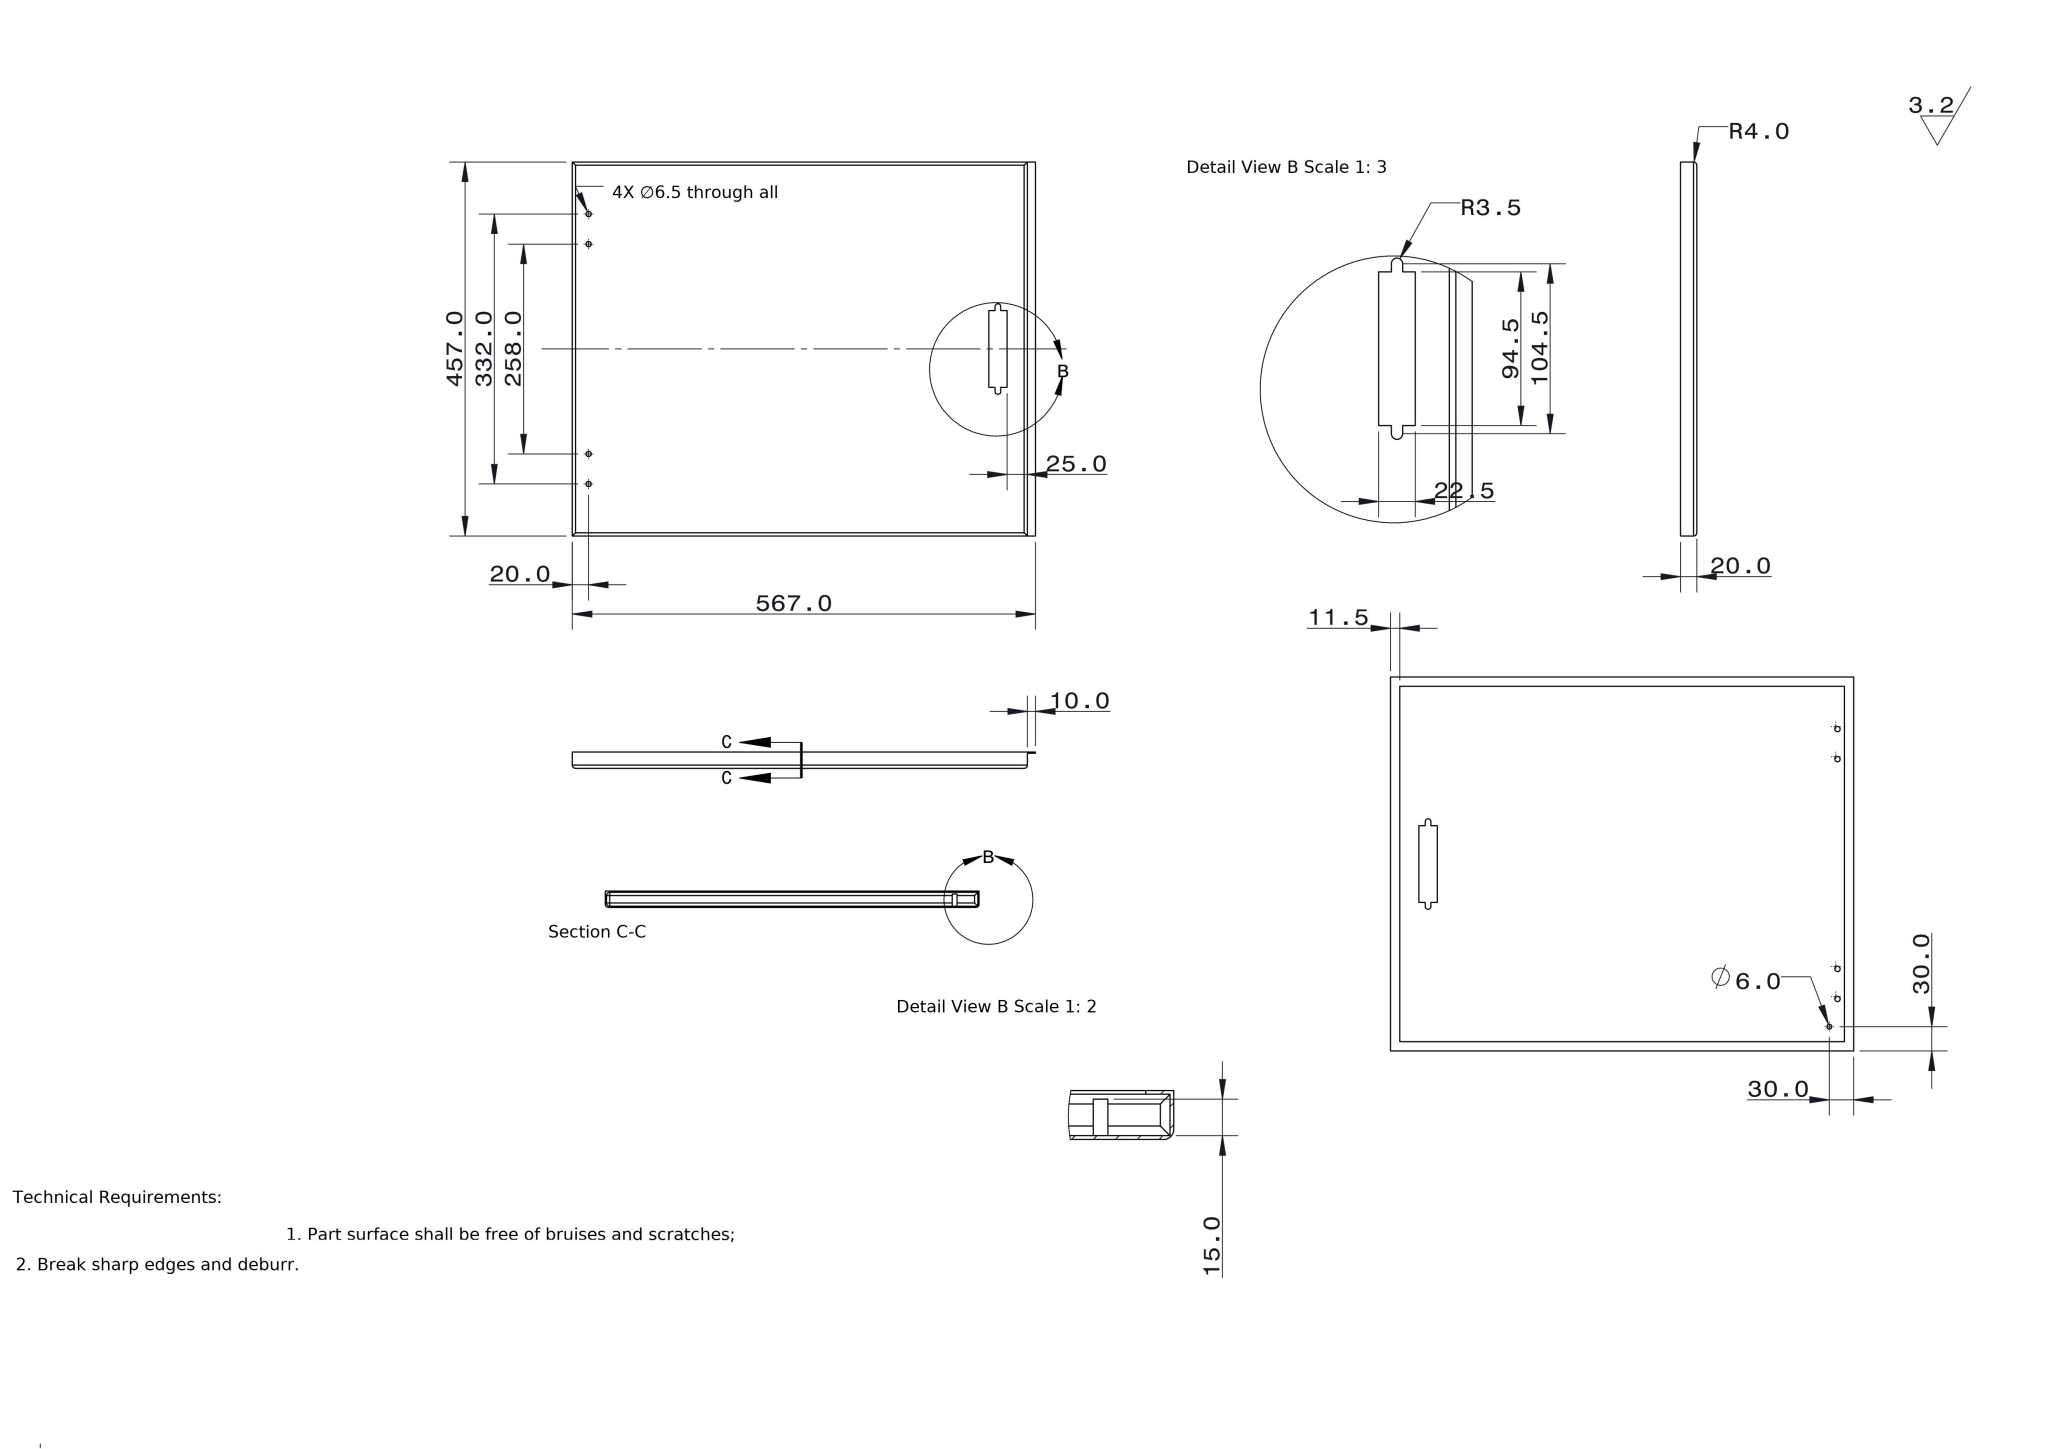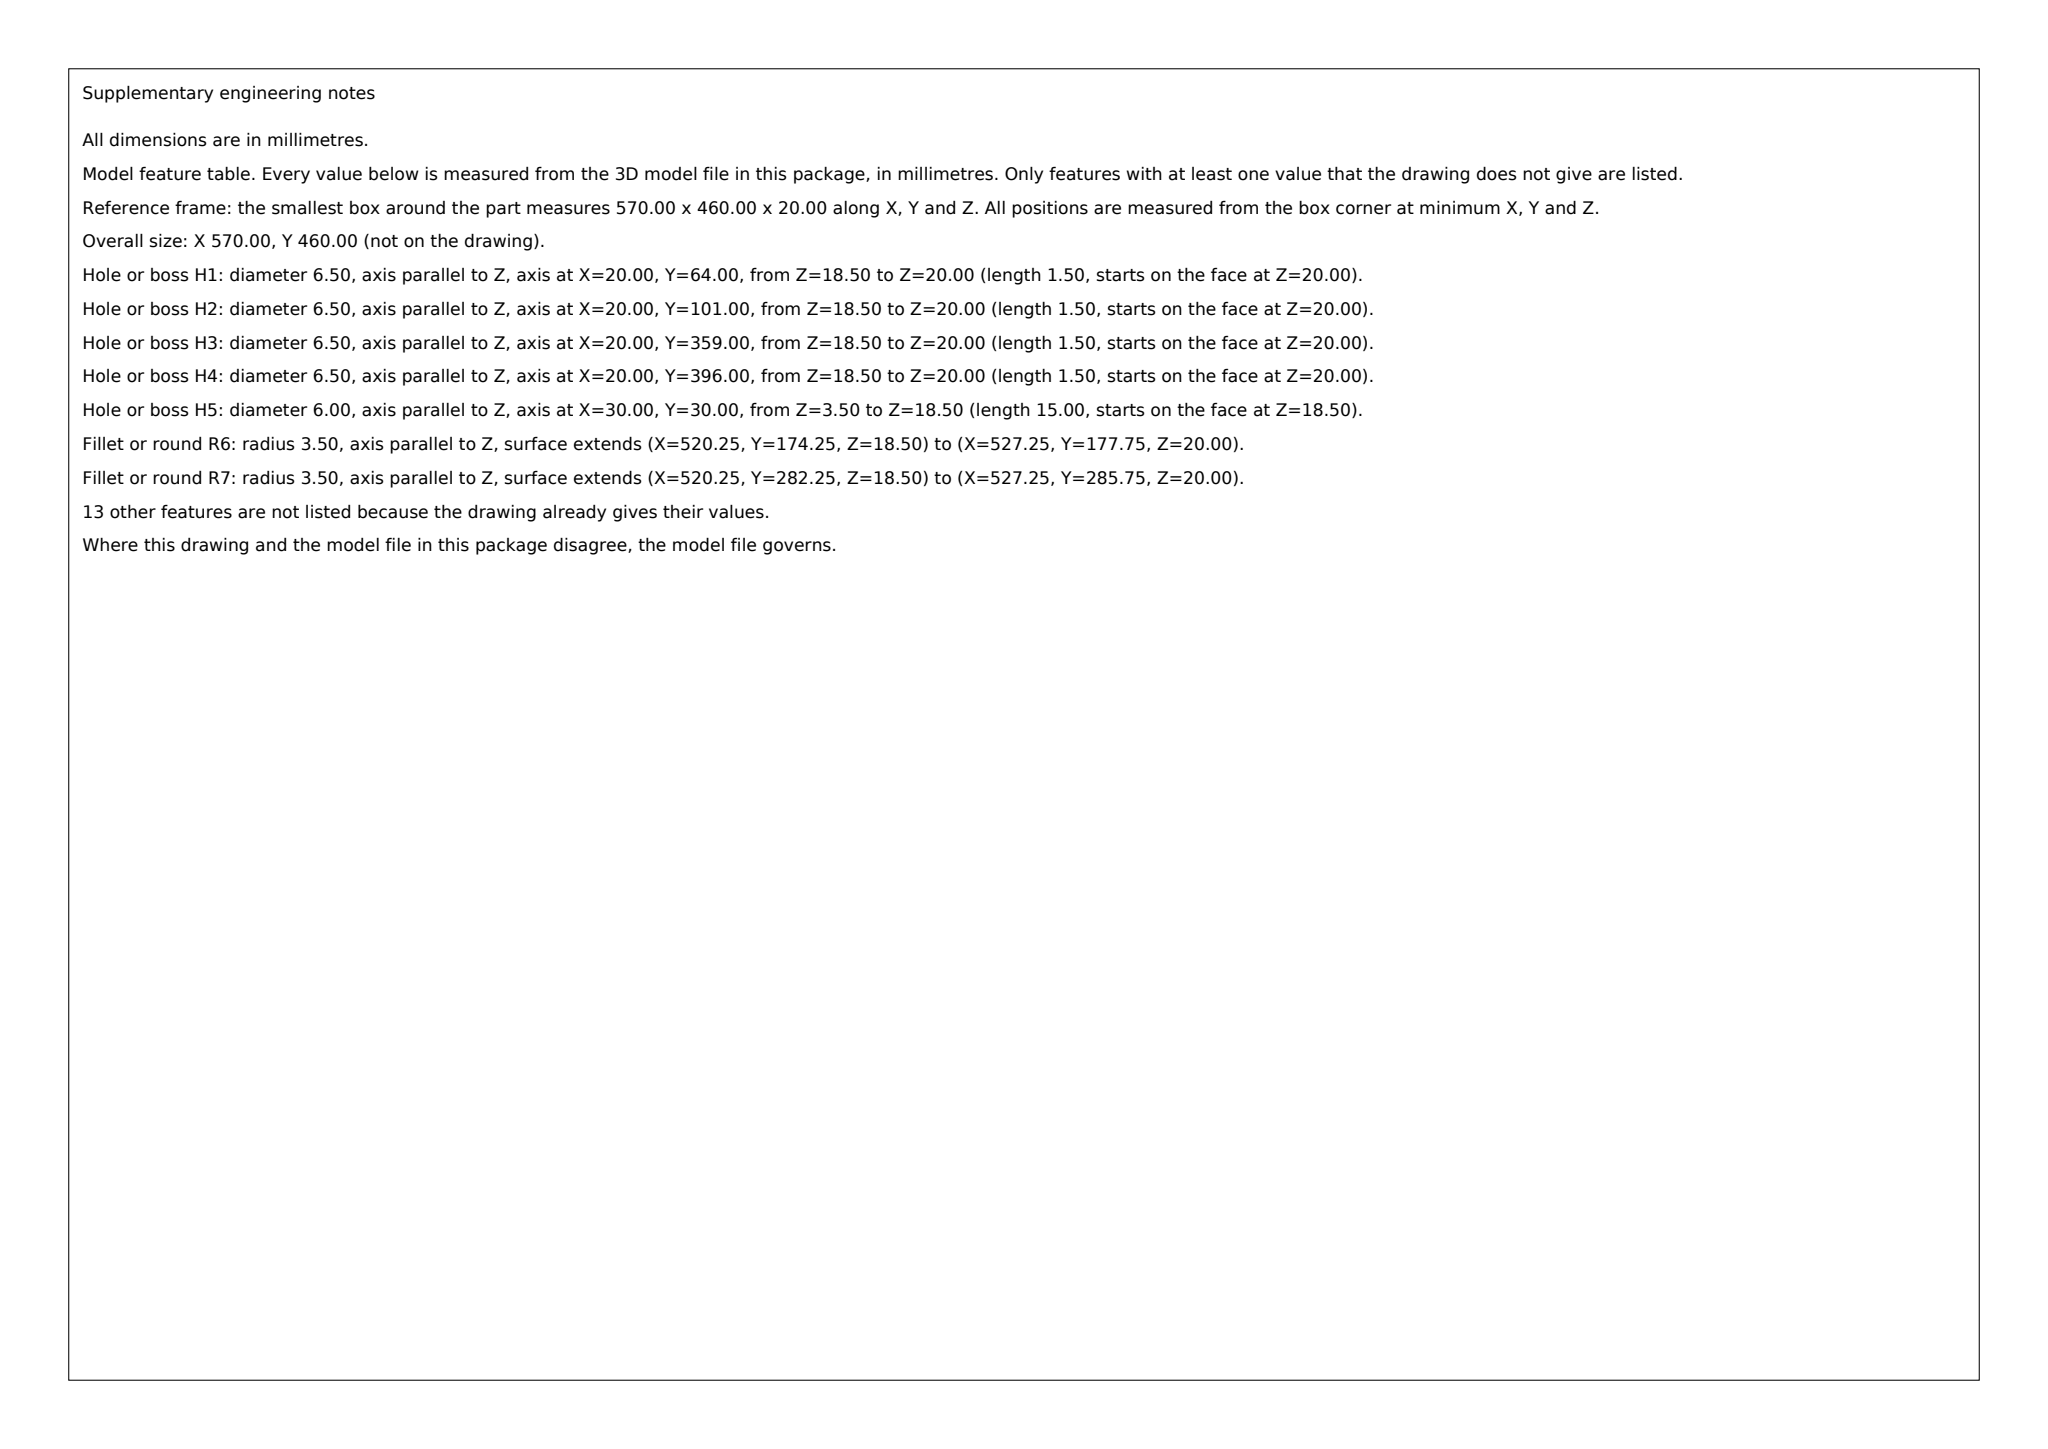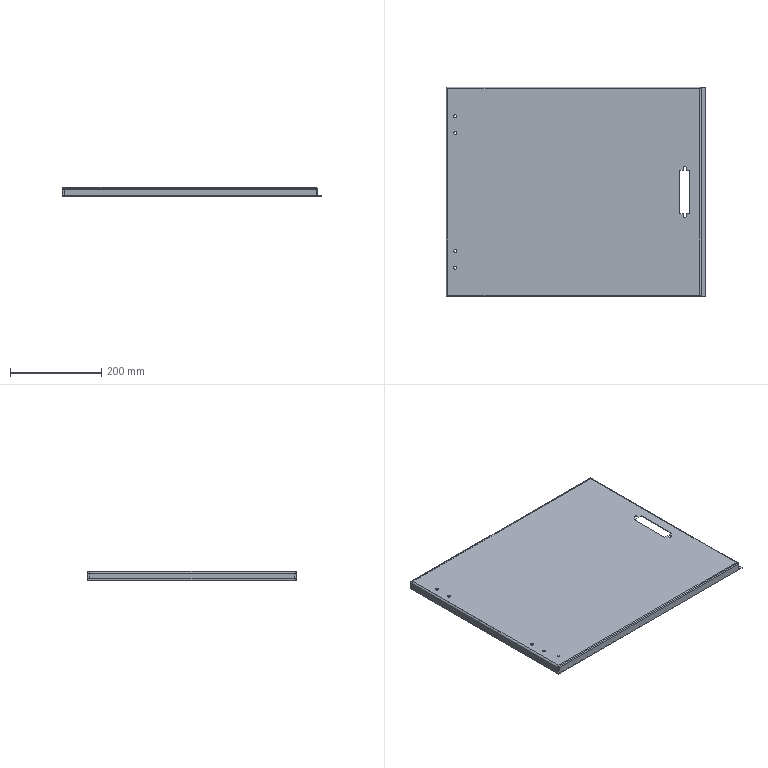Part | SolidWorks | mm | 1 solid | 53 faces | box 570 x 460 x 20 mm | volume 469994 mm3 | plane 28 | cylinder 23 | sphere 2 | commonest cylinder face diameters 8 x11 6.5 x8 6 x2 7 x2
build123d program:
from build123d import *

# Parameters (mm, degrees)
SKETCH1_W                  = 560
SKETCH1_H                  = 460
BOSS_EXTRUDE1_DEPTH        = 20
SHELL1_T                   = -1.5
SKETCH2_W                  = 1.5
SKETCH2_H                  = 460
BOSS_EXTRUDE2_DEPTH        = 10
SKETCH4_W                  = 557
SKETCH4_H                  = 1.5
BOSS_EXTRUDE3_DEPTH        = 10
SKETCH5_W                  = 1.5
SKETCH5_H                  = 447
BOSS_EXTRUDE4_DEPTH        = 10
SKETCH6_W                  = 547
SKETCH6_H                  = 1.5
BOSS_EXTRUDE5_DEPTH        = 10
FILLET1_R                  = 4
SKETCH10_R                 = 3
BOSS_EXTRUDE7_DEPTH        = 15
F_6_5_6_5_DIAMETER_HOLE1_D = 6.5
CUT_EXTRUDE1_DEPTH         = 5105.746


with BuildPart() as part:
    # Sketch1 → Boss-Extrude1 (new body)
    with BuildSketch(Plane.XY):
        with Locations((98.751, 4859.883)):
            Rectangle(SKETCH1_W, SKETCH1_H)
    extrude(amount=BOSS_EXTRUDE1_DEPTH)

    # Shell1
    shell1_openings = [part.faces().sort_by_distance(p)[0] for p in [
        (98.751, 4859.883, 0),
    ]]
    offset(amount=SHELL1_T, openings=shell1_openings, kind=Kind.INTERSECTION)

    # Sketch2 → Boss-Extrude2 (add)
    with BuildSketch(Plane(origin=(378.751, 0, 0), x_dir=(0, 0, -1), z_dir=(1, 0, 0))):
        with Locations((-0.75, 4859.883)):
            Rectangle(SKETCH2_W, SKETCH2_H)
    extrude(amount=BOSS_EXTRUDE2_DEPTH)

    # Sketch4 → Boss-Extrude3 (add)
    with BuildSketch(Plane(origin=(0, 5088.383, 0), x_dir=(-1, 0, 0), z_dir=(0, -1, 0))):
        with Locations((-98.751, -0.75)):
            Rectangle(SKETCH4_W, SKETCH4_H)
    extrude(amount=BOSS_EXTRUDE3_DEPTH)

    # Sketch5 → Boss-Extrude4 (add)
    with BuildSketch(Plane(origin=(-179.749, 0, 0), x_dir=(0, 0, -1), z_dir=(1, 0, 0))):
        with Locations((-0.75, 4854.883)):
            Rectangle(SKETCH5_W, SKETCH5_H)
    extrude(amount=BOSS_EXTRUDE4_DEPTH)

    # Sketch6 → Boss-Extrude5 (add)
    with BuildSketch(Plane(origin=(0, 4631.383, 0), x_dir=(-1, 0, 0), z_dir=(0, 1, 0))):
        with Locations((-103.751, 0.75)):
            Rectangle(SKETCH6_W, SKETCH6_H)
    extrude(amount=BOSS_EXTRUDE5_DEPTH)

    # Fillet1
    fillet1_edges = [part.edges().sort_by_distance(p)[0] for p in [
        (-179.749, 4859.883, 18.5),
        (-179.749, 4859.883, 1.5),
        (-179.749, 4631.383, 10),
        (98.751, 5088.383, 18.5),
        (377.251, 5088.383, 10),
        (98.751, 5088.383, 1.5),
        (-179.749, 5088.383, 10),
        (98.751, 4629.883, 20),
        (-181.249, 4859.883, 20),
        (98.751, 5089.883, 20),
        (378.751, 4859.883, 20),
    ]]
    fillet(fillet1_edges, radius=FILLET1_R)

    # Sketch10 → Boss-Extrude7 (add)
    with BuildSketch(Plane(origin=(0, 0, 18.5), x_dir=(-1, 0, 0), z_dir=(0, 0, -1))):
        with Locations(Location((151.249, 4659.883, 0), (0, 0, 180))):
            Circle(SKETCH10_R)
    extrude(amount=BOSS_EXTRUDE7_DEPTH)

    # 6.5 _6.5_ Diameter Hole1 (through all)
    with Locations(Plane.XY.offset(20)):
        with Locations((-161.249, 5025.883), (-161.249, 4988.883), (-161.249, 4730.883), (-161.249, 4693.883)):
            Hole(F_6_5_6_5_DIAMETER_HOLE1_D / 2)

    # Sketch7 → Cut-Extrude1 (cut, through all)
    with BuildSketch(Plane.XY.offset(20)):
        with BuildLine():
            Line((346.001, 4812.633), (346.001, 4807.633))
            ThreePointArc((346.001, 4807.633), (342.501, 4804.133), (339.001, 4807.633))
            Line((339.001, 4807.633), (339.001, 4812.633))
            Line((339.001, 4812.633), (331.251, 4812.633))
            Line((331.251, 4812.633), (331.251, 4907.133))
            Line((331.251, 4907.133), (339.001, 4907.133))
            Line((339.001, 4907.133), (339.001, 4912.133))
            ThreePointArc((339.001, 4912.133), (342.501, 4915.633), (346.001, 4912.133))
            Line((346.001, 4912.133), (346.001, 4907.133))
            Line((346.001, 4907.133), (353.751, 4907.133))
            Line((353.751, 4907.133), (353.751, 4812.633))
            Line((353.751, 4812.633), (346.001, 4812.633))
        make_face()
    extrude(amount=-CUT_EXTRUDE1_DEPTH, mode=Mode.SUBTRACT)


solid = part.part